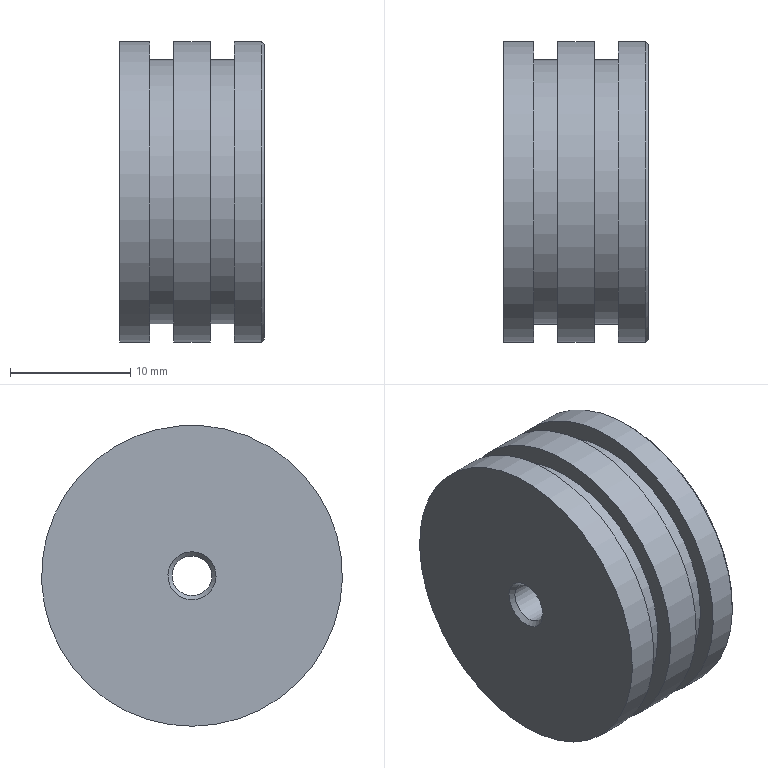Component | NX | PISTON | 1 solid | 15 faces | box 12 x 25 x 25 mm | volume 5341 mm3 | plane 6 | cylinder 6 | cone 3 | commonest cylinder face diameters 25 x3 22 x2 3.3 x1
STEP:
#1=CARTESIAN_POINT('',(0.,0.,0.));
#2=DIRECTION('',(0.,0.,1.));
#3=DIRECTION('',(1.,0.,0.));
#4=AXIS2_PLACEMENT_3D('',#1,#2,#3);
#5=CARTESIAN_POINT('',(408.474,87.539,111.392));
#6=VERTEX_POINT('',#5);
#7=CARTESIAN_POINT('',(408.474,89.5,111.));
#8=DIRECTION('',(1.,0.,0.));
#9=DIRECTION('',(0.,-0.9806,0.1959));
#10=AXIS2_PLACEMENT_3D('',#7,#8,#9);
#11=CIRCLE('',#10,2.);
#12=CARTESIAN_POINT('',(408.474,87.051,98.742));
#13=DIRECTION('',(-1.,0.,0.));
#14=DIRECTION('',(0.,-0.9806,0.1959));
#15=AXIS2_PLACEMENT_3D('',#12,#13,#14);
#16=PLANE('',#15);
#17=CARTESIAN_POINT('',(2.,12.5));
#18=CARTESIAN_POINT('',(2.,9.036));
#19=CARTESIAN_POINT('',(-1.,10.768));
#20=CARTESIAN_POINT('',(-4.,12.5));
#21=CARTESIAN_POINT('',(-1.,14.232));
#22=CARTESIAN_POINT('',(2.,15.964));
#23=CARTESIAN_POINT('',(2.,12.5));
#24=(BOUNDED_CURVE()B_SPLINE_CURVE(2,(#17,#18,#19,#20,#21,#22,#23),.UNSPECIFIED.,.T.,.F.)B_SPLINE_CURVE_WITH_KNOTS((1,2,2,2,2,1),(-2.094,0.,2.094,4.189,6.283,8.378),.UNSPECIFIED.)CURVE()GEOMETRIC_REPRESENTATION_ITEM()RATIONAL_B_SPLINE_CURVE((1.,0.5,1.,0.5,1.,0.5,1.))REPRESENTATION_ITEM(''));
#25=(GEOMETRIC_REPRESENTATION_CONTEXT(2)PARAMETRIC_REPRESENTATION_CONTEXT()REPRESENTATION_CONTEXT('',''));
#26=DEFINITIONAL_REPRESENTATION('',(#24),#25);
#27=PCURVE('',#16,#26);
#28=CARTESIAN_POINT('',(408.824,89.5,111.));
#29=DIRECTION('',(-1.,0.,0.));
#30=DIRECTION('',(0.,-0.9806,0.1959));
#31=AXIS2_PLACEMENT_3D('',#28,#29,#30);
#32=CONICAL_SURFACE('',#31,1.65,0.7854);
#33=CARTESIAN_POINT('',(6.283,0.35));
#34=DIRECTION('',(-1.,0.));
#35=VECTOR('',#34,1.);
#36=LINE('',#33,#35);
#37=(GEOMETRIC_REPRESENTATION_CONTEXT(2)PARAMETRIC_REPRESENTATION_CONTEXT()REPRESENTATION_CONTEXT('',''));
#38=DEFINITIONAL_REPRESENTATION('',(#36),#37);
#39=PCURVE('',#32,#38);
#40=SURFACE_CURVE('',#11,(#27,#39),.PCURVE_S1.);
#41=EDGE_CURVE('',#6,#6,#40,.T.);
#42=ORIENTED_EDGE('',*,*,#41,.T.);
#43=EDGE_LOOP('',(#42));
#44=FACE_BOUND('',#43,.T.);
#45=CARTESIAN_POINT('',(408.474,101.758,108.551));
#46=VERTEX_POINT('',#45);
#47=CARTESIAN_POINT('',(408.474,89.5,111.));
#48=DIRECTION('',(1.,0.,0.));
#49=DIRECTION('',(0.,0.9806,-0.1959));
#50=AXIS2_PLACEMENT_3D('',#47,#48,#49);
#51=CIRCLE('',#50,12.5);
#52=CARTESIAN_POINT('',(-12.5,12.5));
#53=CARTESIAN_POINT('',(-12.5,34.151));
#54=CARTESIAN_POINT('',(6.25,23.325));
#55=CARTESIAN_POINT('',(25.,12.5));
#56=CARTESIAN_POINT('',(6.25,1.675));
#57=CARTESIAN_POINT('',(-12.5,-9.151));
#58=CARTESIAN_POINT('',(-12.5,12.5));
#59=(BOUNDED_CURVE()B_SPLINE_CURVE(2,(#52,#53,#54,#55,#56,#57,#58),.UNSPECIFIED.,.T.,.F.)B_SPLINE_CURVE_WITH_KNOTS((1,2,2,2,2,1),(-2.094,0.,2.094,4.189,6.283,8.378),.UNSPECIFIED.)CURVE()GEOMETRIC_REPRESENTATION_ITEM()RATIONAL_B_SPLINE_CURVE((1.,0.5,1.,0.5,1.,0.5,1.))REPRESENTATION_ITEM(''));
#60=(GEOMETRIC_REPRESENTATION_CONTEXT(2)PARAMETRIC_REPRESENTATION_CONTEXT()REPRESENTATION_CONTEXT('',''));
#61=DEFINITIONAL_REPRESENTATION('',(#59),#60);
#62=PCURVE('',#16,#61);
#63=CARTESIAN_POINT('',(408.474,89.5,111.));
#64=DIRECTION('',(1.,0.,0.));
#65=DIRECTION('',(0.,0.9806,-0.1959));
#66=AXIS2_PLACEMENT_3D('',#63,#64,#65);
#67=CYLINDRICAL_SURFACE('',#66,12.5);
#68=CARTESIAN_POINT('',(0.,0.));
#69=DIRECTION('',(1.,0.));
#70=VECTOR('',#69,1.);
#71=LINE('',#68,#70);
#72=(GEOMETRIC_REPRESENTATION_CONTEXT(2)PARAMETRIC_REPRESENTATION_CONTEXT()REPRESENTATION_CONTEXT('',''));
#73=DEFINITIONAL_REPRESENTATION('',(#71),#72);
#74=PCURVE('',#67,#73);
#75=SURFACE_CURVE('',#51,(#62,#74),.PCURVE_S1.);
#76=EDGE_CURVE('',#46,#46,#75,.T.);
#77=ORIENTED_EDGE('',*,*,#76,.F.);
#78=EDGE_LOOP('',(#77));
#79=FACE_BOUND('',#78,.T.);
#80=ADVANCED_FACE('',(#44,#79),#16,.T.);
#81=ORIENTED_EDGE('',*,*,#76,.T.);
#82=CARTESIAN_POINT('',(410.974,101.758,108.551));
#83=VERTEX_POINT('',#82);
#84=CARTESIAN_POINT('',(408.474,101.758,108.551));
#85=CARTESIAN_POINT('',(410.974,101.758,108.551));
#86=B_SPLINE_CURVE_WITH_KNOTS('',1,(#84,#85),.UNSPECIFIED.,.F.,.F.,(2,2),(0.,2.5),.PIECEWISE_BEZIER_KNOTS.);
#87=CARTESIAN_POINT('',(6.283,0.));
#88=DIRECTION('',(0.,1.));
#89=VECTOR('',#88,1.);
#90=LINE('',#87,#89);
#91=(GEOMETRIC_REPRESENTATION_CONTEXT(2)PARAMETRIC_REPRESENTATION_CONTEXT()REPRESENTATION_CONTEXT('',''));
#92=DEFINITIONAL_REPRESENTATION('',(#90),#91);
#93=PCURVE('',#67,#92);
#94=CARTESIAN_POINT('',(0.,0.));
#95=DIRECTION('',(0.,1.));
#96=VECTOR('',#95,1.);
#97=LINE('',#94,#96);
#98=(GEOMETRIC_REPRESENTATION_CONTEXT(2)PARAMETRIC_REPRESENTATION_CONTEXT()REPRESENTATION_CONTEXT('',''));
#99=DEFINITIONAL_REPRESENTATION('',(#97),#98);
#100=PCURVE('',#67,#99);
#101=SEAM_CURVE('',#86,(#93,#100),.PCURVE_S1.);
#102=EDGE_CURVE('',#46,#83,#101,.T.);
#103=ORIENTED_EDGE('',*,*,#102,.T.);
#104=CARTESIAN_POINT('',(410.974,89.5,111.));
#105=DIRECTION('',(1.,0.,0.));
#106=DIRECTION('',(0.,0.9806,-0.1959));
#107=AXIS2_PLACEMENT_3D('',#104,#105,#106);
#108=CIRCLE('',#107,12.5);
#109=CARTESIAN_POINT('',(0.,2.5));
#110=DIRECTION('',(1.,0.));
#111=VECTOR('',#110,1.);
#112=LINE('',#109,#111);
#113=(GEOMETRIC_REPRESENTATION_CONTEXT(2)PARAMETRIC_REPRESENTATION_CONTEXT()REPRESENTATION_CONTEXT('',''));
#114=DEFINITIONAL_REPRESENTATION('',(#112),#113);
#115=PCURVE('',#67,#114);
#116=CARTESIAN_POINT('',(410.974,87.345,100.213));
#117=DIRECTION('',(1.,0.,0.));
#118=DIRECTION('',(0.,0.9806,-0.1959));
#119=AXIS2_PLACEMENT_3D('',#116,#117,#118);
#120=PLANE('',#119);
#121=CARTESIAN_POINT('',(0.,11.));
#122=DIRECTION('',(1.,0.));
#123=AXIS2_PLACEMENT_2D('',#121,#122);
#124=CIRCLE('',#123,12.5);
#125=(GEOMETRIC_REPRESENTATION_CONTEXT(2)PARAMETRIC_REPRESENTATION_CONTEXT()REPRESENTATION_CONTEXT('',''));
#126=DEFINITIONAL_REPRESENTATION('',(#124),#125);
#127=PCURVE('',#120,#126);
#128=SURFACE_CURVE('',#108,(#115,#127),.PCURVE_S1.);
#129=EDGE_CURVE('',#83,#83,#128,.T.);
#130=ORIENTED_EDGE('',*,*,#129,.F.);
#131=ORIENTED_EDGE('',*,*,#102,.F.);
#132=EDGE_LOOP('',(#81,#103,#130,#131));
#133=FACE_BOUND('',#132,.T.);
#134=ADVANCED_FACE('',(#133),#67,.T.);
#135=ORIENTED_EDGE('',*,*,#129,.T.);
#136=EDGE_LOOP('',(#135));
#137=FACE_BOUND('',#136,.T.);
#138=CARTESIAN_POINT('',(410.974,100.287,108.845));
#139=VERTEX_POINT('',#138);
#140=CARTESIAN_POINT('',(410.974,89.5,111.));
#141=DIRECTION('',(1.,0.,0.));
#142=DIRECTION('',(0.,0.9806,-0.1959));
#143=AXIS2_PLACEMENT_3D('',#140,#141,#142);
#144=CIRCLE('',#143,11.);
#145=CARTESIAN_POINT('',(0.,11.));
#146=DIRECTION('',(1.,0.));
#147=AXIS2_PLACEMENT_2D('',#145,#146);
#148=CIRCLE('',#147,11.);
#149=(GEOMETRIC_REPRESENTATION_CONTEXT(2)PARAMETRIC_REPRESENTATION_CONTEXT()REPRESENTATION_CONTEXT('',''));
#150=DEFINITIONAL_REPRESENTATION('',(#148),#149);
#151=PCURVE('',#120,#150);
#152=CARTESIAN_POINT('',(408.474,89.5,111.));
#153=DIRECTION('',(1.,0.,0.));
#154=DIRECTION('',(0.,0.9806,-0.1959));
#155=AXIS2_PLACEMENT_3D('',#152,#153,#154);
#156=CYLINDRICAL_SURFACE('',#155,11.);
#157=CARTESIAN_POINT('',(0.,2.5));
#158=DIRECTION('',(1.,0.));
#159=VECTOR('',#158,1.);
#160=LINE('',#157,#159);
#161=(GEOMETRIC_REPRESENTATION_CONTEXT(2)PARAMETRIC_REPRESENTATION_CONTEXT()REPRESENTATION_CONTEXT('',''));
#162=DEFINITIONAL_REPRESENTATION('',(#160),#161);
#163=PCURVE('',#156,#162);
#164=SURFACE_CURVE('',#144,(#151,#163),.PCURVE_S1.);
#165=EDGE_CURVE('',#139,#139,#164,.T.);
#166=ORIENTED_EDGE('',*,*,#165,.F.);
#167=EDGE_LOOP('',(#166));
#168=FACE_BOUND('',#167,.T.);
#169=ADVANCED_FACE('',(#137,#168),#120,.T.);
#170=ORIENTED_EDGE('',*,*,#165,.T.);
#171=CARTESIAN_POINT('',(412.974,100.287,108.845));
#172=VERTEX_POINT('',#171);
#173=CARTESIAN_POINT('',(410.974,100.287,108.845));
#174=CARTESIAN_POINT('',(412.974,100.287,108.845));
#175=B_SPLINE_CURVE_WITH_KNOTS('',1,(#173,#174),.UNSPECIFIED.,.F.,.F.,(2,2),(2.5,4.5),.PIECEWISE_BEZIER_KNOTS.);
#176=CARTESIAN_POINT('',(6.283,0.));
#177=DIRECTION('',(0.,1.));
#178=VECTOR('',#177,1.);
#179=LINE('',#176,#178);
#180=(GEOMETRIC_REPRESENTATION_CONTEXT(2)PARAMETRIC_REPRESENTATION_CONTEXT()REPRESENTATION_CONTEXT('',''));
#181=DEFINITIONAL_REPRESENTATION('',(#179),#180);
#182=PCURVE('',#156,#181);
#183=CARTESIAN_POINT('',(0.,0.));
#184=DIRECTION('',(0.,1.));
#185=VECTOR('',#184,1.);
#186=LINE('',#183,#185);
#187=(GEOMETRIC_REPRESENTATION_CONTEXT(2)PARAMETRIC_REPRESENTATION_CONTEXT()REPRESENTATION_CONTEXT('',''));
#188=DEFINITIONAL_REPRESENTATION('',(#186),#187);
#189=PCURVE('',#156,#188);
#190=SEAM_CURVE('',#175,(#182,#189),.PCURVE_S1.);
#191=EDGE_CURVE('',#139,#172,#190,.T.);
#192=ORIENTED_EDGE('',*,*,#191,.T.);
#193=CARTESIAN_POINT('',(412.974,89.5,111.));
#194=DIRECTION('',(1.,0.,0.));
#195=DIRECTION('',(0.,0.9806,-0.1959));
#196=AXIS2_PLACEMENT_3D('',#193,#194,#195);
#197=CIRCLE('',#196,11.);
#198=CARTESIAN_POINT('',(0.,4.5));
#199=DIRECTION('',(1.,0.));
#200=VECTOR('',#199,1.);
#201=LINE('',#198,#200);
#202=(GEOMETRIC_REPRESENTATION_CONTEXT(2)PARAMETRIC_REPRESENTATION_CONTEXT()REPRESENTATION_CONTEXT('',''));
#203=DEFINITIONAL_REPRESENTATION('',(#201),#202);
#204=PCURVE('',#156,#203);
#205=CARTESIAN_POINT('',(412.974,87.051,98.742));
#206=DIRECTION('',(-1.,0.,0.));
#207=DIRECTION('',(0.,-0.9806,0.1959));
#208=AXIS2_PLACEMENT_3D('',#205,#206,#207);
#209=PLANE('',#208);
#210=CARTESIAN_POINT('',(-11.,12.5));
#211=CARTESIAN_POINT('',(-11.,31.553));
#212=CARTESIAN_POINT('',(5.5,22.026));
#213=CARTESIAN_POINT('',(22.,12.5));
#214=CARTESIAN_POINT('',(5.5,2.974));
#215=CARTESIAN_POINT('',(-11.,-6.553));
#216=CARTESIAN_POINT('',(-11.,12.5));
#217=(BOUNDED_CURVE()B_SPLINE_CURVE(2,(#210,#211,#212,#213,#214,#215,#216),.UNSPECIFIED.,.T.,.F.)B_SPLINE_CURVE_WITH_KNOTS((1,2,2,2,2,1),(-2.094,0.,2.094,4.189,6.283,8.378),.UNSPECIFIED.)CURVE()GEOMETRIC_REPRESENTATION_ITEM()RATIONAL_B_SPLINE_CURVE((1.,0.5,1.,0.5,1.,0.5,1.))REPRESENTATION_ITEM(''));
#218=(GEOMETRIC_REPRESENTATION_CONTEXT(2)PARAMETRIC_REPRESENTATION_CONTEXT()REPRESENTATION_CONTEXT('',''));
#219=DEFINITIONAL_REPRESENTATION('',(#217),#218);
#220=PCURVE('',#209,#219);
#221=SURFACE_CURVE('',#197,(#204,#220),.PCURVE_S1.);
#222=EDGE_CURVE('',#172,#172,#221,.T.);
#223=ORIENTED_EDGE('',*,*,#222,.F.);
#224=ORIENTED_EDGE('',*,*,#191,.F.);
#225=EDGE_LOOP('',(#170,#192,#223,#224));
#226=FACE_BOUND('',#225,.T.);
#227=ADVANCED_FACE('',(#226),#156,.T.);
#228=ORIENTED_EDGE('',*,*,#222,.T.);
#229=EDGE_LOOP('',(#228));
#230=FACE_BOUND('',#229,.T.);
#231=CARTESIAN_POINT('',(412.974,101.758,108.551));
#232=VERTEX_POINT('',#231);
#233=CARTESIAN_POINT('',(412.974,89.5,111.));
#234=DIRECTION('',(1.,0.,0.));
#235=DIRECTION('',(0.,0.9806,-0.1959));
#236=AXIS2_PLACEMENT_3D('',#233,#234,#235);
#237=CIRCLE('',#236,12.5);
#238=CARTESIAN_POINT('',(-12.5,12.5));
#239=CARTESIAN_POINT('',(-12.5,34.151));
#240=CARTESIAN_POINT('',(6.25,23.325));
#241=CARTESIAN_POINT('',(25.,12.5));
#242=CARTESIAN_POINT('',(6.25,1.675));
#243=CARTESIAN_POINT('',(-12.5,-9.151));
#244=CARTESIAN_POINT('',(-12.5,12.5));
#245=(BOUNDED_CURVE()B_SPLINE_CURVE(2,(#238,#239,#240,#241,#242,#243,#244),.UNSPECIFIED.,.T.,.F.)B_SPLINE_CURVE_WITH_KNOTS((1,2,2,2,2,1),(-2.094,0.,2.094,4.189,6.283,8.378),.UNSPECIFIED.)CURVE()GEOMETRIC_REPRESENTATION_ITEM()RATIONAL_B_SPLINE_CURVE((1.,0.5,1.,0.5,1.,0.5,1.))REPRESENTATION_ITEM(''));
#246=(GEOMETRIC_REPRESENTATION_CONTEXT(2)PARAMETRIC_REPRESENTATION_CONTEXT()REPRESENTATION_CONTEXT('',''));
#247=DEFINITIONAL_REPRESENTATION('',(#245),#246);
#248=PCURVE('',#209,#247);
#249=CARTESIAN_POINT('',(408.474,89.5,111.));
#250=DIRECTION('',(1.,0.,0.));
#251=DIRECTION('',(0.,0.9806,-0.1959));
#252=AXIS2_PLACEMENT_3D('',#249,#250,#251);
#253=CYLINDRICAL_SURFACE('',#252,12.5);
#254=CARTESIAN_POINT('',(0.,4.5));
#255=DIRECTION('',(1.,0.));
#256=VECTOR('',#255,1.);
#257=LINE('',#254,#256);
#258=(GEOMETRIC_REPRESENTATION_CONTEXT(2)PARAMETRIC_REPRESENTATION_CONTEXT()REPRESENTATION_CONTEXT('',''));
#259=DEFINITIONAL_REPRESENTATION('',(#257),#258);
#260=PCURVE('',#253,#259);
#261=SURFACE_CURVE('',#237,(#248,#260),.PCURVE_S1.);
#262=EDGE_CURVE('',#232,#232,#261,.T.);
#263=ORIENTED_EDGE('',*,*,#262,.F.);
#264=EDGE_LOOP('',(#263));
#265=FACE_BOUND('',#264,.T.);
#266=ADVANCED_FACE('',(#230,#265),#209,.T.);
#267=ORIENTED_EDGE('',*,*,#262,.T.);
#268=CARTESIAN_POINT('',(415.974,101.758,108.551));
#269=VERTEX_POINT('',#268);
#270=CARTESIAN_POINT('',(412.974,101.758,108.551));
#271=CARTESIAN_POINT('',(415.974,101.758,108.551));
#272=B_SPLINE_CURVE_WITH_KNOTS('',1,(#270,#271),.UNSPECIFIED.,.F.,.F.,(2,2),(4.5,7.5),.PIECEWISE_BEZIER_KNOTS.);
#273=CARTESIAN_POINT('',(6.283,0.));
#274=DIRECTION('',(0.,1.));
#275=VECTOR('',#274,1.);
#276=LINE('',#273,#275);
#277=(GEOMETRIC_REPRESENTATION_CONTEXT(2)PARAMETRIC_REPRESENTATION_CONTEXT()REPRESENTATION_CONTEXT('',''));
#278=DEFINITIONAL_REPRESENTATION('',(#276),#277);
#279=PCURVE('',#253,#278);
#280=CARTESIAN_POINT('',(0.,0.));
#281=DIRECTION('',(0.,1.));
#282=VECTOR('',#281,1.);
#283=LINE('',#280,#282);
#284=(GEOMETRIC_REPRESENTATION_CONTEXT(2)PARAMETRIC_REPRESENTATION_CONTEXT()REPRESENTATION_CONTEXT('',''));
#285=DEFINITIONAL_REPRESENTATION('',(#283),#284);
#286=PCURVE('',#253,#285);
#287=SEAM_CURVE('',#272,(#279,#286),.PCURVE_S1.);
#288=EDGE_CURVE('',#232,#269,#287,.T.);
#289=ORIENTED_EDGE('',*,*,#288,.T.);
#290=CARTESIAN_POINT('',(415.974,89.5,111.));
#291=DIRECTION('',(1.,0.,0.));
#292=DIRECTION('',(0.,0.9806,-0.1959));
#293=AXIS2_PLACEMENT_3D('',#290,#291,#292);
#294=CIRCLE('',#293,12.5);
#295=CARTESIAN_POINT('',(0.,7.5));
#296=DIRECTION('',(1.,0.));
#297=VECTOR('',#296,1.);
#298=LINE('',#295,#297);
#299=(GEOMETRIC_REPRESENTATION_CONTEXT(2)PARAMETRIC_REPRESENTATION_CONTEXT()REPRESENTATION_CONTEXT('',''));
#300=DEFINITIONAL_REPRESENTATION('',(#298),#299);
#301=PCURVE('',#253,#300);
#302=CARTESIAN_POINT('',(415.974,87.345,100.213));
#303=DIRECTION('',(1.,0.,0.));
#304=DIRECTION('',(0.,0.9806,-0.1959));
#305=AXIS2_PLACEMENT_3D('',#302,#303,#304);
#306=PLANE('',#305);
#307=CARTESIAN_POINT('',(0.,11.));
#308=DIRECTION('',(1.,0.));
#309=AXIS2_PLACEMENT_2D('',#307,#308);
#310=CIRCLE('',#309,12.5);
#311=(GEOMETRIC_REPRESENTATION_CONTEXT(2)PARAMETRIC_REPRESENTATION_CONTEXT()REPRESENTATION_CONTEXT('',''));
#312=DEFINITIONAL_REPRESENTATION('',(#310),#311);
#313=PCURVE('',#306,#312);
#314=SURFACE_CURVE('',#294,(#301,#313),.PCURVE_S1.);
#315=EDGE_CURVE('',#269,#269,#314,.T.);
#316=ORIENTED_EDGE('',*,*,#315,.F.);
#317=ORIENTED_EDGE('',*,*,#288,.F.);
#318=EDGE_LOOP('',(#267,#289,#316,#317));
#319=FACE_BOUND('',#318,.T.);
#320=ADVANCED_FACE('',(#319),#253,.T.);
#321=ORIENTED_EDGE('',*,*,#315,.T.);
#322=EDGE_LOOP('',(#321));
#323=FACE_BOUND('',#322,.T.);
#324=CARTESIAN_POINT('',(415.974,100.287,108.845));
#325=VERTEX_POINT('',#324);
#326=CARTESIAN_POINT('',(415.974,89.5,111.));
#327=DIRECTION('',(1.,0.,0.));
#328=DIRECTION('',(0.,0.9806,-0.1959));
#329=AXIS2_PLACEMENT_3D('',#326,#327,#328);
#330=CIRCLE('',#329,11.);
#331=CARTESIAN_POINT('',(0.,11.));
#332=DIRECTION('',(1.,0.));
#333=AXIS2_PLACEMENT_2D('',#331,#332);
#334=CIRCLE('',#333,11.);
#335=(GEOMETRIC_REPRESENTATION_CONTEXT(2)PARAMETRIC_REPRESENTATION_CONTEXT()REPRESENTATION_CONTEXT('',''));
#336=DEFINITIONAL_REPRESENTATION('',(#334),#335);
#337=PCURVE('',#306,#336);
#338=CARTESIAN_POINT('',(408.474,89.5,111.));
#339=DIRECTION('',(1.,0.,0.));
#340=DIRECTION('',(0.,0.9806,-0.1959));
#341=AXIS2_PLACEMENT_3D('',#338,#339,#340);
#342=CYLINDRICAL_SURFACE('',#341,11.);
#343=CARTESIAN_POINT('',(0.,7.5));
#344=DIRECTION('',(1.,0.));
#345=VECTOR('',#344,1.);
#346=LINE('',#343,#345);
#347=(GEOMETRIC_REPRESENTATION_CONTEXT(2)PARAMETRIC_REPRESENTATION_CONTEXT()REPRESENTATION_CONTEXT('',''));
#348=DEFINITIONAL_REPRESENTATION('',(#346),#347);
#349=PCURVE('',#342,#348);
#350=SURFACE_CURVE('',#330,(#337,#349),.PCURVE_S1.);
#351=EDGE_CURVE('',#325,#325,#350,.T.);
#352=ORIENTED_EDGE('',*,*,#351,.F.);
#353=EDGE_LOOP('',(#352));
#354=FACE_BOUND('',#353,.T.);
#355=ADVANCED_FACE('',(#323,#354),#306,.T.);
#356=ORIENTED_EDGE('',*,*,#351,.T.);
#357=CARTESIAN_POINT('',(417.974,100.287,108.845));
#358=VERTEX_POINT('',#357);
#359=CARTESIAN_POINT('',(415.974,100.287,108.845));
#360=CARTESIAN_POINT('',(417.974,100.287,108.845));
#361=B_SPLINE_CURVE_WITH_KNOTS('',1,(#359,#360),.UNSPECIFIED.,.F.,.F.,(2,2),(7.5,9.5),.PIECEWISE_BEZIER_KNOTS.);
#362=CARTESIAN_POINT('',(6.283,0.));
#363=DIRECTION('',(0.,1.));
#364=VECTOR('',#363,1.);
#365=LINE('',#362,#364);
#366=(GEOMETRIC_REPRESENTATION_CONTEXT(2)PARAMETRIC_REPRESENTATION_CONTEXT()REPRESENTATION_CONTEXT('',''));
#367=DEFINITIONAL_REPRESENTATION('',(#365),#366);
#368=PCURVE('',#342,#367);
#369=CARTESIAN_POINT('',(0.,0.));
#370=DIRECTION('',(0.,1.));
#371=VECTOR('',#370,1.);
#372=LINE('',#369,#371);
#373=(GEOMETRIC_REPRESENTATION_CONTEXT(2)PARAMETRIC_REPRESENTATION_CONTEXT()REPRESENTATION_CONTEXT('',''));
#374=DEFINITIONAL_REPRESENTATION('',(#372),#373);
#375=PCURVE('',#342,#374);
#376=SEAM_CURVE('',#361,(#368,#375),.PCURVE_S1.);
#377=EDGE_CURVE('',#325,#358,#376,.T.);
#378=ORIENTED_EDGE('',*,*,#377,.T.);
#379=CARTESIAN_POINT('',(417.974,89.5,111.));
#380=DIRECTION('',(1.,0.,0.));
#381=DIRECTION('',(0.,0.9806,-0.1959));
#382=AXIS2_PLACEMENT_3D('',#379,#380,#381);
#383=CIRCLE('',#382,11.);
#384=CARTESIAN_POINT('',(0.,9.5));
#385=DIRECTION('',(1.,0.));
#386=VECTOR('',#385,1.);
#387=LINE('',#384,#386);
#388=(GEOMETRIC_REPRESENTATION_CONTEXT(2)PARAMETRIC_REPRESENTATION_CONTEXT()REPRESENTATION_CONTEXT('',''));
#389=DEFINITIONAL_REPRESENTATION('',(#387),#388);
#390=PCURVE('',#342,#389);
#391=CARTESIAN_POINT('',(417.974,87.051,98.742));
#392=DIRECTION('',(-1.,0.,0.));
#393=DIRECTION('',(0.,-0.9806,0.1959));
#394=AXIS2_PLACEMENT_3D('',#391,#392,#393);
#395=PLANE('',#394);
#396=CARTESIAN_POINT('',(-11.,12.5));
#397=CARTESIAN_POINT('',(-11.,31.553));
#398=CARTESIAN_POINT('',(5.5,22.026));
#399=CARTESIAN_POINT('',(22.,12.5));
#400=CARTESIAN_POINT('',(5.5,2.974));
#401=CARTESIAN_POINT('',(-11.,-6.553));
#402=CARTESIAN_POINT('',(-11.,12.5));
#403=(BOUNDED_CURVE()B_SPLINE_CURVE(2,(#396,#397,#398,#399,#400,#401,#402),.UNSPECIFIED.,.T.,.F.)B_SPLINE_CURVE_WITH_KNOTS((1,2,2,2,2,1),(-2.094,0.,2.094,4.189,6.283,8.378),.UNSPECIFIED.)CURVE()GEOMETRIC_REPRESENTATION_ITEM()RATIONAL_B_SPLINE_CURVE((1.,0.5,1.,0.5,1.,0.5,1.))REPRESENTATION_ITEM(''));
#404=(GEOMETRIC_REPRESENTATION_CONTEXT(2)PARAMETRIC_REPRESENTATION_CONTEXT()REPRESENTATION_CONTEXT('',''));
#405=DEFINITIONAL_REPRESENTATION('',(#403),#404);
#406=PCURVE('',#395,#405);
#407=SURFACE_CURVE('',#383,(#390,#406),.PCURVE_S1.);
#408=EDGE_CURVE('',#358,#358,#407,.T.);
#409=ORIENTED_EDGE('',*,*,#408,.F.);
#410=ORIENTED_EDGE('',*,*,#377,.F.);
#411=EDGE_LOOP('',(#356,#378,#409,#410));
#412=FACE_BOUND('',#411,.T.);
#413=ADVANCED_FACE('',(#412),#342,.T.);
#414=ORIENTED_EDGE('',*,*,#408,.T.);
#415=EDGE_LOOP('',(#414));
#416=FACE_BOUND('',#415,.T.);
#417=CARTESIAN_POINT('',(417.974,101.758,108.551));
#418=VERTEX_POINT('',#417);
#419=CARTESIAN_POINT('',(417.974,89.5,111.));
#420=DIRECTION('',(1.,0.,0.));
#421=DIRECTION('',(0.,0.9806,-0.1959));
#422=AXIS2_PLACEMENT_3D('',#419,#420,#421);
#423=CIRCLE('',#422,12.5);
#424=CARTESIAN_POINT('',(-12.5,12.5));
#425=CARTESIAN_POINT('',(-12.5,34.151));
#426=CARTESIAN_POINT('',(6.25,23.325));
#427=CARTESIAN_POINT('',(25.,12.5));
#428=CARTESIAN_POINT('',(6.25,1.675));
#429=CARTESIAN_POINT('',(-12.5,-9.151));
#430=CARTESIAN_POINT('',(-12.5,12.5));
#431=(BOUNDED_CURVE()B_SPLINE_CURVE(2,(#424,#425,#426,#427,#428,#429,#430),.UNSPECIFIED.,.T.,.F.)B_SPLINE_CURVE_WITH_KNOTS((1,2,2,2,2,1),(-2.094,0.,2.094,4.189,6.283,8.378),.UNSPECIFIED.)CURVE()GEOMETRIC_REPRESENTATION_ITEM()RATIONAL_B_SPLINE_CURVE((1.,0.5,1.,0.5,1.,0.5,1.))REPRESENTATION_ITEM(''));
#432=(GEOMETRIC_REPRESENTATION_CONTEXT(2)PARAMETRIC_REPRESENTATION_CONTEXT()REPRESENTATION_CONTEXT('',''));
#433=DEFINITIONAL_REPRESENTATION('',(#431),#432);
#434=PCURVE('',#395,#433);
#435=CARTESIAN_POINT('',(408.474,89.5,111.));
#436=DIRECTION('',(1.,0.,0.));
#437=DIRECTION('',(0.,0.9806,-0.1959));
#438=AXIS2_PLACEMENT_3D('',#435,#436,#437);
#439=CYLINDRICAL_SURFACE('',#438,12.5);
#440=CARTESIAN_POINT('',(0.,9.5));
#441=DIRECTION('',(1.,0.));
#442=VECTOR('',#441,1.);
#443=LINE('',#440,#442);
#444=(GEOMETRIC_REPRESENTATION_CONTEXT(2)PARAMETRIC_REPRESENTATION_CONTEXT()REPRESENTATION_CONTEXT('',''));
#445=DEFINITIONAL_REPRESENTATION('',(#443),#444);
#446=PCURVE('',#439,#445);
#447=SURFACE_CURVE('',#423,(#434,#446),.PCURVE_S1.);
#448=EDGE_CURVE('',#418,#418,#447,.T.);
#449=ORIENTED_EDGE('',*,*,#448,.F.);
#450=EDGE_LOOP('',(#449));
#451=FACE_BOUND('',#450,.T.);
#452=ADVANCED_FACE('',(#416,#451),#395,.T.);
#453=CARTESIAN_POINT('',(420.224,101.758,108.551));
#454=VERTEX_POINT('',#453);
#455=CARTESIAN_POINT('',(420.224,89.5,111.));
#456=DIRECTION('',(-1.,0.,0.));
#457=DIRECTION('',(0.,0.9806,-0.1959));
#458=AXIS2_PLACEMENT_3D('',#455,#456,#457);
#459=CIRCLE('',#458,12.5);
#460=CARTESIAN_POINT('',(6.283,11.75));
#461=DIRECTION('',(-1.,0.));
#462=VECTOR('',#461,1.);
#463=LINE('',#460,#462);
#464=(GEOMETRIC_REPRESENTATION_CONTEXT(2)PARAMETRIC_REPRESENTATION_CONTEXT()REPRESENTATION_CONTEXT('',''));
#465=DEFINITIONAL_REPRESENTATION('',(#463),#464);
#466=PCURVE('',#439,#465);
#467=CARTESIAN_POINT('',(420.474,89.5,111.));
#468=DIRECTION('',(-1.,0.,0.));
#469=DIRECTION('',(0.,-0.9806,0.1959));
#470=AXIS2_PLACEMENT_3D('',#467,#468,#469);
#471=CONICAL_SURFACE('',#470,12.25,0.7854);
#472=CARTESIAN_POINT('',(3.142,0.25));
#473=DIRECTION('',(1.,0.));
#474=VECTOR('',#473,1.);
#475=LINE('',#472,#474);
#476=(GEOMETRIC_REPRESENTATION_CONTEXT(2)PARAMETRIC_REPRESENTATION_CONTEXT()REPRESENTATION_CONTEXT('',''));
#477=DEFINITIONAL_REPRESENTATION('',(#475),#476);
#478=PCURVE('',#471,#477);
#479=SURFACE_CURVE('',#459,(#466,#478),.PCURVE_S1.);
#480=EDGE_CURVE('',#454,#454,#479,.T.);
#481=ORIENTED_EDGE('',*,*,#480,.T.);
#482=CARTESIAN_POINT('',(417.974,101.758,108.551));
#483=CARTESIAN_POINT('',(420.224,101.758,108.551));
#484=B_SPLINE_CURVE_WITH_KNOTS('',1,(#482,#483),.UNSPECIFIED.,.F.,.F.,(2,2),(9.5,11.75),.PIECEWISE_BEZIER_KNOTS.);
#485=CARTESIAN_POINT('',(0.,0.));
#486=DIRECTION('',(0.,1.));
#487=VECTOR('',#486,1.);
#488=LINE('',#485,#487);
#489=(GEOMETRIC_REPRESENTATION_CONTEXT(2)PARAMETRIC_REPRESENTATION_CONTEXT()REPRESENTATION_CONTEXT('',''));
#490=DEFINITIONAL_REPRESENTATION('',(#488),#489);
#491=PCURVE('',#439,#490);
#492=CARTESIAN_POINT('',(6.283,0.));
#493=DIRECTION('',(0.,1.));
#494=VECTOR('',#493,1.);
#495=LINE('',#492,#494);
#496=(GEOMETRIC_REPRESENTATION_CONTEXT(2)PARAMETRIC_REPRESENTATION_CONTEXT()REPRESENTATION_CONTEXT('',''));
#497=DEFINITIONAL_REPRESENTATION('',(#495),#496);
#498=PCURVE('',#439,#497);
#499=SEAM_CURVE('',#484,(#491,#498),.PCURVE_S1.);
#500=EDGE_CURVE('',#418,#454,#499,.T.);
#501=ORIENTED_EDGE('',*,*,#500,.F.);
#502=ORIENTED_EDGE('',*,*,#448,.T.);
#503=ORIENTED_EDGE('',*,*,#500,.T.);
#504=EDGE_LOOP('',(#481,#501,#502,#503));
#505=FACE_BOUND('',#504,.T.);
#506=ADVANCED_FACE('',(#505),#439,.T.);
#507=CARTESIAN_POINT('',(420.474,101.513,108.6));
#508=VERTEX_POINT('',#507);
#509=CARTESIAN_POINT('',(420.474,89.5,111.));
#510=DIRECTION('',(1.,0.,0.));
#511=DIRECTION('',(0.,0.9806,-0.1959));
#512=AXIS2_PLACEMENT_3D('',#509,#510,#511);
#513=CIRCLE('',#512,12.25);
#514=CARTESIAN_POINT('',(420.474,89.5,111.));
#515=DIRECTION('',(1.,0.,0.));
#516=DIRECTION('',(0.,0.9806,-0.1959));
#517=AXIS2_PLACEMENT_3D('',#514,#515,#516);
#518=PLANE('',#517);
#519=CARTESIAN_POINT('',(0.,0.));
#520=DIRECTION('',(1.,0.));
#521=AXIS2_PLACEMENT_2D('',#519,#520);
#522=CIRCLE('',#521,12.25);
#523=(GEOMETRIC_REPRESENTATION_CONTEXT(2)PARAMETRIC_REPRESENTATION_CONTEXT()REPRESENTATION_CONTEXT('',''));
#524=DEFINITIONAL_REPRESENTATION('',(#522),#523);
#525=PCURVE('',#518,#524);
#526=CARTESIAN_POINT('',(9.425,0.));
#527=DIRECTION('',(-1.,0.));
#528=VECTOR('',#527,1.);
#529=LINE('',#526,#528);
#530=(GEOMETRIC_REPRESENTATION_CONTEXT(2)PARAMETRIC_REPRESENTATION_CONTEXT()REPRESENTATION_CONTEXT('',''));
#531=DEFINITIONAL_REPRESENTATION('',(#529),#530);
#532=PCURVE('',#471,#531);
#533=SURFACE_CURVE('',#513,(#525,#532),.PCURVE_S1.);
#534=EDGE_CURVE('',#508,#508,#533,.T.);
#535=ORIENTED_EDGE('',*,*,#534,.T.);
#536=EDGE_LOOP('',(#535));
#537=FACE_BOUND('',#536,.T.);
#538=CARTESIAN_POINT('',(420.474,91.461,110.608));
#539=VERTEX_POINT('',#538);
#540=CARTESIAN_POINT('',(420.474,89.5,111.));
#541=DIRECTION('',(-1.,0.,0.));
#542=DIRECTION('',(0.,0.9806,-0.1959));
#543=AXIS2_PLACEMENT_3D('',#540,#541,#542);
#544=CIRCLE('',#543,2.);
#545=CARTESIAN_POINT('',(2.,0.));
#546=CARTESIAN_POINT('',(2.,-3.464));
#547=CARTESIAN_POINT('',(-1.,-1.732));
#548=CARTESIAN_POINT('',(-4.,-0.));
#549=CARTESIAN_POINT('',(-1.,1.732));
#550=CARTESIAN_POINT('',(2.,3.464));
#551=CARTESIAN_POINT('',(2.,0.));
#552=(BOUNDED_CURVE()B_SPLINE_CURVE(2,(#545,#546,#547,#548,#549,#550,#551),.UNSPECIFIED.,.T.,.F.)B_SPLINE_CURVE_WITH_KNOTS((1,2,2,2,2,1),(-2.094,0.,2.094,4.189,6.283,8.378),.UNSPECIFIED.)CURVE()GEOMETRIC_REPRESENTATION_ITEM()RATIONAL_B_SPLINE_CURVE((1.,0.5,1.,0.5,1.,0.5,1.))REPRESENTATION_ITEM(''));
#553=(GEOMETRIC_REPRESENTATION_CONTEXT(2)PARAMETRIC_REPRESENTATION_CONTEXT()REPRESENTATION_CONTEXT('',''));
#554=DEFINITIONAL_REPRESENTATION('',(#552),#553);
#555=PCURVE('',#518,#554);
#556=CARTESIAN_POINT('',(420.474,89.5,111.));
#557=DIRECTION('',(1.,0.,0.));
#558=DIRECTION('',(0.,0.9806,-0.1959));
#559=AXIS2_PLACEMENT_3D('',#556,#557,#558);
#560=CONICAL_SURFACE('',#559,2.,0.7854);
#561=CARTESIAN_POINT('',(6.283,0.));
#562=DIRECTION('',(-1.,0.));
#563=VECTOR('',#562,1.);
#564=LINE('',#561,#563);
#565=(GEOMETRIC_REPRESENTATION_CONTEXT(2)PARAMETRIC_REPRESENTATION_CONTEXT()REPRESENTATION_CONTEXT('',''));
#566=DEFINITIONAL_REPRESENTATION('',(#564),#565);
#567=PCURVE('',#560,#566);
#568=SURFACE_CURVE('',#544,(#555,#567),.PCURVE_S1.);
#569=EDGE_CURVE('',#539,#539,#568,.T.);
#570=ORIENTED_EDGE('',*,*,#569,.T.);
#571=EDGE_LOOP('',(#570));
#572=FACE_BOUND('',#571,.T.);
#573=ADVANCED_FACE('',(#537,#572),#518,.T.);
#574=CARTESIAN_POINT('',(408.824,87.882,111.323));
#575=VERTEX_POINT('',#574);
#576=CARTESIAN_POINT('',(408.824,89.5,111.));
#577=DIRECTION('',(-1.,0.,0.));
#578=DIRECTION('',(0.,-0.9806,0.1959));
#579=AXIS2_PLACEMENT_3D('',#576,#577,#578);
#580=CIRCLE('',#579,1.65);
#581=CARTESIAN_POINT('',(420.474,89.5,111.));
#582=DIRECTION('',(-1.,0.,0.));
#583=DIRECTION('',(0.,-0.9806,0.1959));
#584=AXIS2_PLACEMENT_3D('',#581,#582,#583);
#585=CYLINDRICAL_SURFACE('',#584,1.65);
#586=CARTESIAN_POINT('',(0.,11.65));
#587=DIRECTION('',(1.,0.));
#588=VECTOR('',#587,1.);
#589=LINE('',#586,#588);
#590=(GEOMETRIC_REPRESENTATION_CONTEXT(2)PARAMETRIC_REPRESENTATION_CONTEXT()REPRESENTATION_CONTEXT('',''));
#591=DEFINITIONAL_REPRESENTATION('',(#589),#590);
#592=PCURVE('',#585,#591);
#593=CARTESIAN_POINT('',(0.,-0.));
#594=DIRECTION('',(1.,0.));
#595=VECTOR('',#594,1.);
#596=LINE('',#593,#595);
#597=(GEOMETRIC_REPRESENTATION_CONTEXT(2)PARAMETRIC_REPRESENTATION_CONTEXT()REPRESENTATION_CONTEXT('',''));
#598=DEFINITIONAL_REPRESENTATION('',(#596),#597);
#599=PCURVE('',#32,#598);
#600=SURFACE_CURVE('',#580,(#592,#599),.PCURVE_S1.);
#601=EDGE_CURVE('',#575,#575,#600,.T.);
#602=ORIENTED_EDGE('',*,*,#601,.F.);
#603=CARTESIAN_POINT('',(420.124,87.882,111.323));
#604=VERTEX_POINT('',#603);
#605=CARTESIAN_POINT('',(420.124,87.882,111.323));
#606=CARTESIAN_POINT('',(408.824,87.882,111.323));
#607=B_SPLINE_CURVE_WITH_KNOTS('',1,(#605,#606),.UNSPECIFIED.,.F.,.F.,(2,2),(0.35,11.65),.PIECEWISE_BEZIER_KNOTS.);
#608=CARTESIAN_POINT('',(0.,0.));
#609=DIRECTION('',(0.,1.));
#610=VECTOR('',#609,1.);
#611=LINE('',#608,#610);
#612=(GEOMETRIC_REPRESENTATION_CONTEXT(2)PARAMETRIC_REPRESENTATION_CONTEXT()REPRESENTATION_CONTEXT('',''));
#613=DEFINITIONAL_REPRESENTATION('',(#611),#612);
#614=PCURVE('',#585,#613);
#615=CARTESIAN_POINT('',(6.283,0.));
#616=DIRECTION('',(0.,1.));
#617=VECTOR('',#616,1.);
#618=LINE('',#615,#617);
#619=(GEOMETRIC_REPRESENTATION_CONTEXT(2)PARAMETRIC_REPRESENTATION_CONTEXT()REPRESENTATION_CONTEXT('',''));
#620=DEFINITIONAL_REPRESENTATION('',(#618),#619);
#621=PCURVE('',#585,#620);
#622=SEAM_CURVE('',#607,(#614,#621),.PCURVE_S1.);
#623=EDGE_CURVE('',#604,#575,#622,.T.);
#624=ORIENTED_EDGE('',*,*,#623,.F.);
#625=CARTESIAN_POINT('',(420.124,91.118,110.677));
#626=VERTEX_POINT('',#625);
#627=CARTESIAN_POINT('',(420.124,89.5,111.));
#628=DIRECTION('',(1.,0.,0.));
#629=DIRECTION('',(0.,0.9806,-0.1959));
#630=AXIS2_PLACEMENT_3D('',#627,#628,#629);
#631=CIRCLE('',#630,1.65);
#632=CARTESIAN_POINT('',(3.142,0.35));
#633=DIRECTION('',(-1.,0.));
#634=VECTOR('',#633,1.);
#635=LINE('',#632,#634);
#636=(GEOMETRIC_REPRESENTATION_CONTEXT(2)PARAMETRIC_REPRESENTATION_CONTEXT()REPRESENTATION_CONTEXT('',''));
#637=DEFINITIONAL_REPRESENTATION('',(#635),#636);
#638=PCURVE('',#585,#637);
#639=CARTESIAN_POINT('',(0.,-0.35));
#640=DIRECTION('',(1.,-0.));
#641=VECTOR('',#640,1.);
#642=LINE('',#639,#641);
#643=(GEOMETRIC_REPRESENTATION_CONTEXT(2)PARAMETRIC_REPRESENTATION_CONTEXT()REPRESENTATION_CONTEXT('',''));
#644=DEFINITIONAL_REPRESENTATION('',(#642),#643);
#645=PCURVE('',#560,#644);
#646=SURFACE_CURVE('',#631,(#638,#645),.PCURVE_S1.);
#647=EDGE_CURVE('',#626,#604,#646,.T.);
#648=ORIENTED_EDGE('',*,*,#647,.F.);
#649=CARTESIAN_POINT('',(420.124,89.5,111.));
#650=DIRECTION('',(1.,0.,0.));
#651=DIRECTION('',(0.,0.9806,-0.1959));
#652=AXIS2_PLACEMENT_3D('',#649,#650,#651);
#653=CIRCLE('',#652,1.65);
#654=CARTESIAN_POINT('',(9.425,0.35));
#655=DIRECTION('',(-1.,0.));
#656=VECTOR('',#655,1.);
#657=LINE('',#654,#656);
#658=(GEOMETRIC_REPRESENTATION_CONTEXT(2)PARAMETRIC_REPRESENTATION_CONTEXT()REPRESENTATION_CONTEXT('',''));
#659=DEFINITIONAL_REPRESENTATION('',(#657),#658);
#660=PCURVE('',#585,#659);
#661=CARTESIAN_POINT('',(0.,-0.35));
#662=DIRECTION('',(1.,0.));
#663=VECTOR('',#662,1.);
#664=LINE('',#661,#663);
#665=(GEOMETRIC_REPRESENTATION_CONTEXT(2)PARAMETRIC_REPRESENTATION_CONTEXT()REPRESENTATION_CONTEXT('',''));
#666=DEFINITIONAL_REPRESENTATION('',(#664),#665);
#667=PCURVE('',#560,#666);
#668=SURFACE_CURVE('',#653,(#660,#667),.PCURVE_S1.);
#669=EDGE_CURVE('',#604,#626,#668,.T.);
#670=ORIENTED_EDGE('',*,*,#669,.F.);
#671=ORIENTED_EDGE('',*,*,#623,.T.);
#672=EDGE_LOOP('',(#602,#624,#648,#670,#671));
#673=FACE_BOUND('',#672,.F.);
#674=ADVANCED_FACE('',(#673),#585,.F.);
#675=ORIENTED_EDGE('',*,*,#669,.T.);
#676=CARTESIAN_POINT('',(420.124,91.118,110.677));
#677=CARTESIAN_POINT('',(420.474,91.461,110.608));
#678=B_SPLINE_CURVE_WITH_KNOTS('',1,(#676,#677),.UNSPECIFIED.,.F.,.F.,(2,2),(-0.495,0.),.PIECEWISE_BEZIER_KNOTS.);
#679=CARTESIAN_POINT('',(6.283,0.));
#680=DIRECTION('',(0.,1.));
#681=VECTOR('',#680,1.);
#682=LINE('',#679,#681);
#683=(GEOMETRIC_REPRESENTATION_CONTEXT(2)PARAMETRIC_REPRESENTATION_CONTEXT()REPRESENTATION_CONTEXT('',''));
#684=DEFINITIONAL_REPRESENTATION('',(#682),#683);
#685=PCURVE('',#560,#684);
#686=CARTESIAN_POINT('',(0.,0.));
#687=DIRECTION('',(0.,1.));
#688=VECTOR('',#687,1.);
#689=LINE('',#686,#688);
#690=(GEOMETRIC_REPRESENTATION_CONTEXT(2)PARAMETRIC_REPRESENTATION_CONTEXT()REPRESENTATION_CONTEXT('',''));
#691=DEFINITIONAL_REPRESENTATION('',(#689),#690);
#692=PCURVE('',#560,#691);
#693=SEAM_CURVE('',#678,(#685,#692),.PCURVE_S1.);
#694=EDGE_CURVE('',#626,#539,#693,.T.);
#695=ORIENTED_EDGE('',*,*,#694,.T.);
#696=ORIENTED_EDGE('',*,*,#569,.T.);
#697=ORIENTED_EDGE('',*,*,#694,.F.);
#698=ORIENTED_EDGE('',*,*,#647,.T.);
#699=EDGE_LOOP('',(#675,#695,#696,#697,#698));
#700=FACE_BOUND('',#699,.F.);
#701=ADVANCED_FACE('',(#700),#560,.F.);
#702=ORIENTED_EDGE('',*,*,#41,.T.);
#703=CARTESIAN_POINT('',(408.824,87.882,111.323));
#704=CARTESIAN_POINT('',(408.474,87.539,111.392));
#705=B_SPLINE_CURVE_WITH_KNOTS('',1,(#703,#704),.UNSPECIFIED.,.F.,.F.,(2,2),(-0.,0.495),.PIECEWISE_BEZIER_KNOTS.);
#706=CARTESIAN_POINT('',(0.,0.));
#707=DIRECTION('',(0.,1.));
#708=VECTOR('',#707,1.);
#709=LINE('',#706,#708);
#710=(GEOMETRIC_REPRESENTATION_CONTEXT(2)PARAMETRIC_REPRESENTATION_CONTEXT()REPRESENTATION_CONTEXT('',''));
#711=DEFINITIONAL_REPRESENTATION('',(#709),#710);
#712=PCURVE('',#32,#711);
#713=CARTESIAN_POINT('',(6.283,0.));
#714=DIRECTION('',(0.,1.));
#715=VECTOR('',#714,1.);
#716=LINE('',#713,#715);
#717=(GEOMETRIC_REPRESENTATION_CONTEXT(2)PARAMETRIC_REPRESENTATION_CONTEXT()REPRESENTATION_CONTEXT('',''));
#718=DEFINITIONAL_REPRESENTATION('',(#716),#717);
#719=PCURVE('',#32,#718);
#720=SEAM_CURVE('',#705,(#712,#719),.PCURVE_S1.);
#721=EDGE_CURVE('',#575,#6,#720,.T.);
#722=ORIENTED_EDGE('',*,*,#721,.F.);
#723=ORIENTED_EDGE('',*,*,#601,.T.);
#724=ORIENTED_EDGE('',*,*,#721,.T.);
#725=EDGE_LOOP('',(#702,#722,#723,#724));
#726=FACE_BOUND('',#725,.F.);
#727=ADVANCED_FACE('',(#726),#32,.F.);
#728=ORIENTED_EDGE('',*,*,#480,.F.);
#729=CARTESIAN_POINT('',(420.474,101.513,108.6));
#730=CARTESIAN_POINT('',(420.224,101.758,108.551));
#731=B_SPLINE_CURVE_WITH_KNOTS('',1,(#729,#730),.UNSPECIFIED.,.F.,.F.,(2,2),(0.,0.3536),.PIECEWISE_BEZIER_KNOTS.);
#732=CARTESIAN_POINT('',(3.142,0.));
#733=DIRECTION('',(0.,1.));
#734=VECTOR('',#733,1.);
#735=LINE('',#732,#734);
#736=(GEOMETRIC_REPRESENTATION_CONTEXT(2)PARAMETRIC_REPRESENTATION_CONTEXT()REPRESENTATION_CONTEXT('',''));
#737=DEFINITIONAL_REPRESENTATION('',(#735),#736);
#738=PCURVE('',#471,#737);
#739=CARTESIAN_POINT('',(9.425,0.));
#740=DIRECTION('',(0.,1.));
#741=VECTOR('',#740,1.);
#742=LINE('',#739,#741);
#743=(GEOMETRIC_REPRESENTATION_CONTEXT(2)PARAMETRIC_REPRESENTATION_CONTEXT()REPRESENTATION_CONTEXT('',''));
#744=DEFINITIONAL_REPRESENTATION('',(#742),#743);
#745=PCURVE('',#471,#744);
#746=SEAM_CURVE('',#731,(#738,#745),.PCURVE_S1.);
#747=EDGE_CURVE('',#508,#454,#746,.T.);
#748=ORIENTED_EDGE('',*,*,#747,.F.);
#749=ORIENTED_EDGE('',*,*,#534,.F.);
#750=ORIENTED_EDGE('',*,*,#747,.T.);
#751=EDGE_LOOP('',(#728,#748,#749,#750));
#752=FACE_BOUND('',#751,.T.);
#753=ADVANCED_FACE('',(#752),#471,.T.);
#754=CLOSED_SHELL('',(#80,#134,#169,#227,#266,#320,#355,#413,#452,#506,#573,#674,#701,#727,#753));
#755=MANIFOLD_SOLID_BREP('',#754);
#756=(LENGTH_UNIT()NAMED_UNIT(*)SI_UNIT(.MILLI.,.METRE.));
#757=UNCERTAINTY_MEASURE_WITH_UNIT(LENGTH_MEASURE(0.00001),#756,'','');
#758=(NAMED_UNIT(*)PLANE_ANGLE_UNIT()SI_UNIT($,.RADIAN.));
#759=(NAMED_UNIT(*)SI_UNIT($,.STERADIAN.)SOLID_ANGLE_UNIT());
#760=(GEOMETRIC_REPRESENTATION_CONTEXT(3)GLOBAL_UNCERTAINTY_ASSIGNED_CONTEXT((#757))GLOBAL_UNIT_ASSIGNED_CONTEXT((#756,#758,#759))REPRESENTATION_CONTEXT('',''));
#761=ADVANCED_BREP_SHAPE_REPRESENTATION('',(#4,#755),#760);